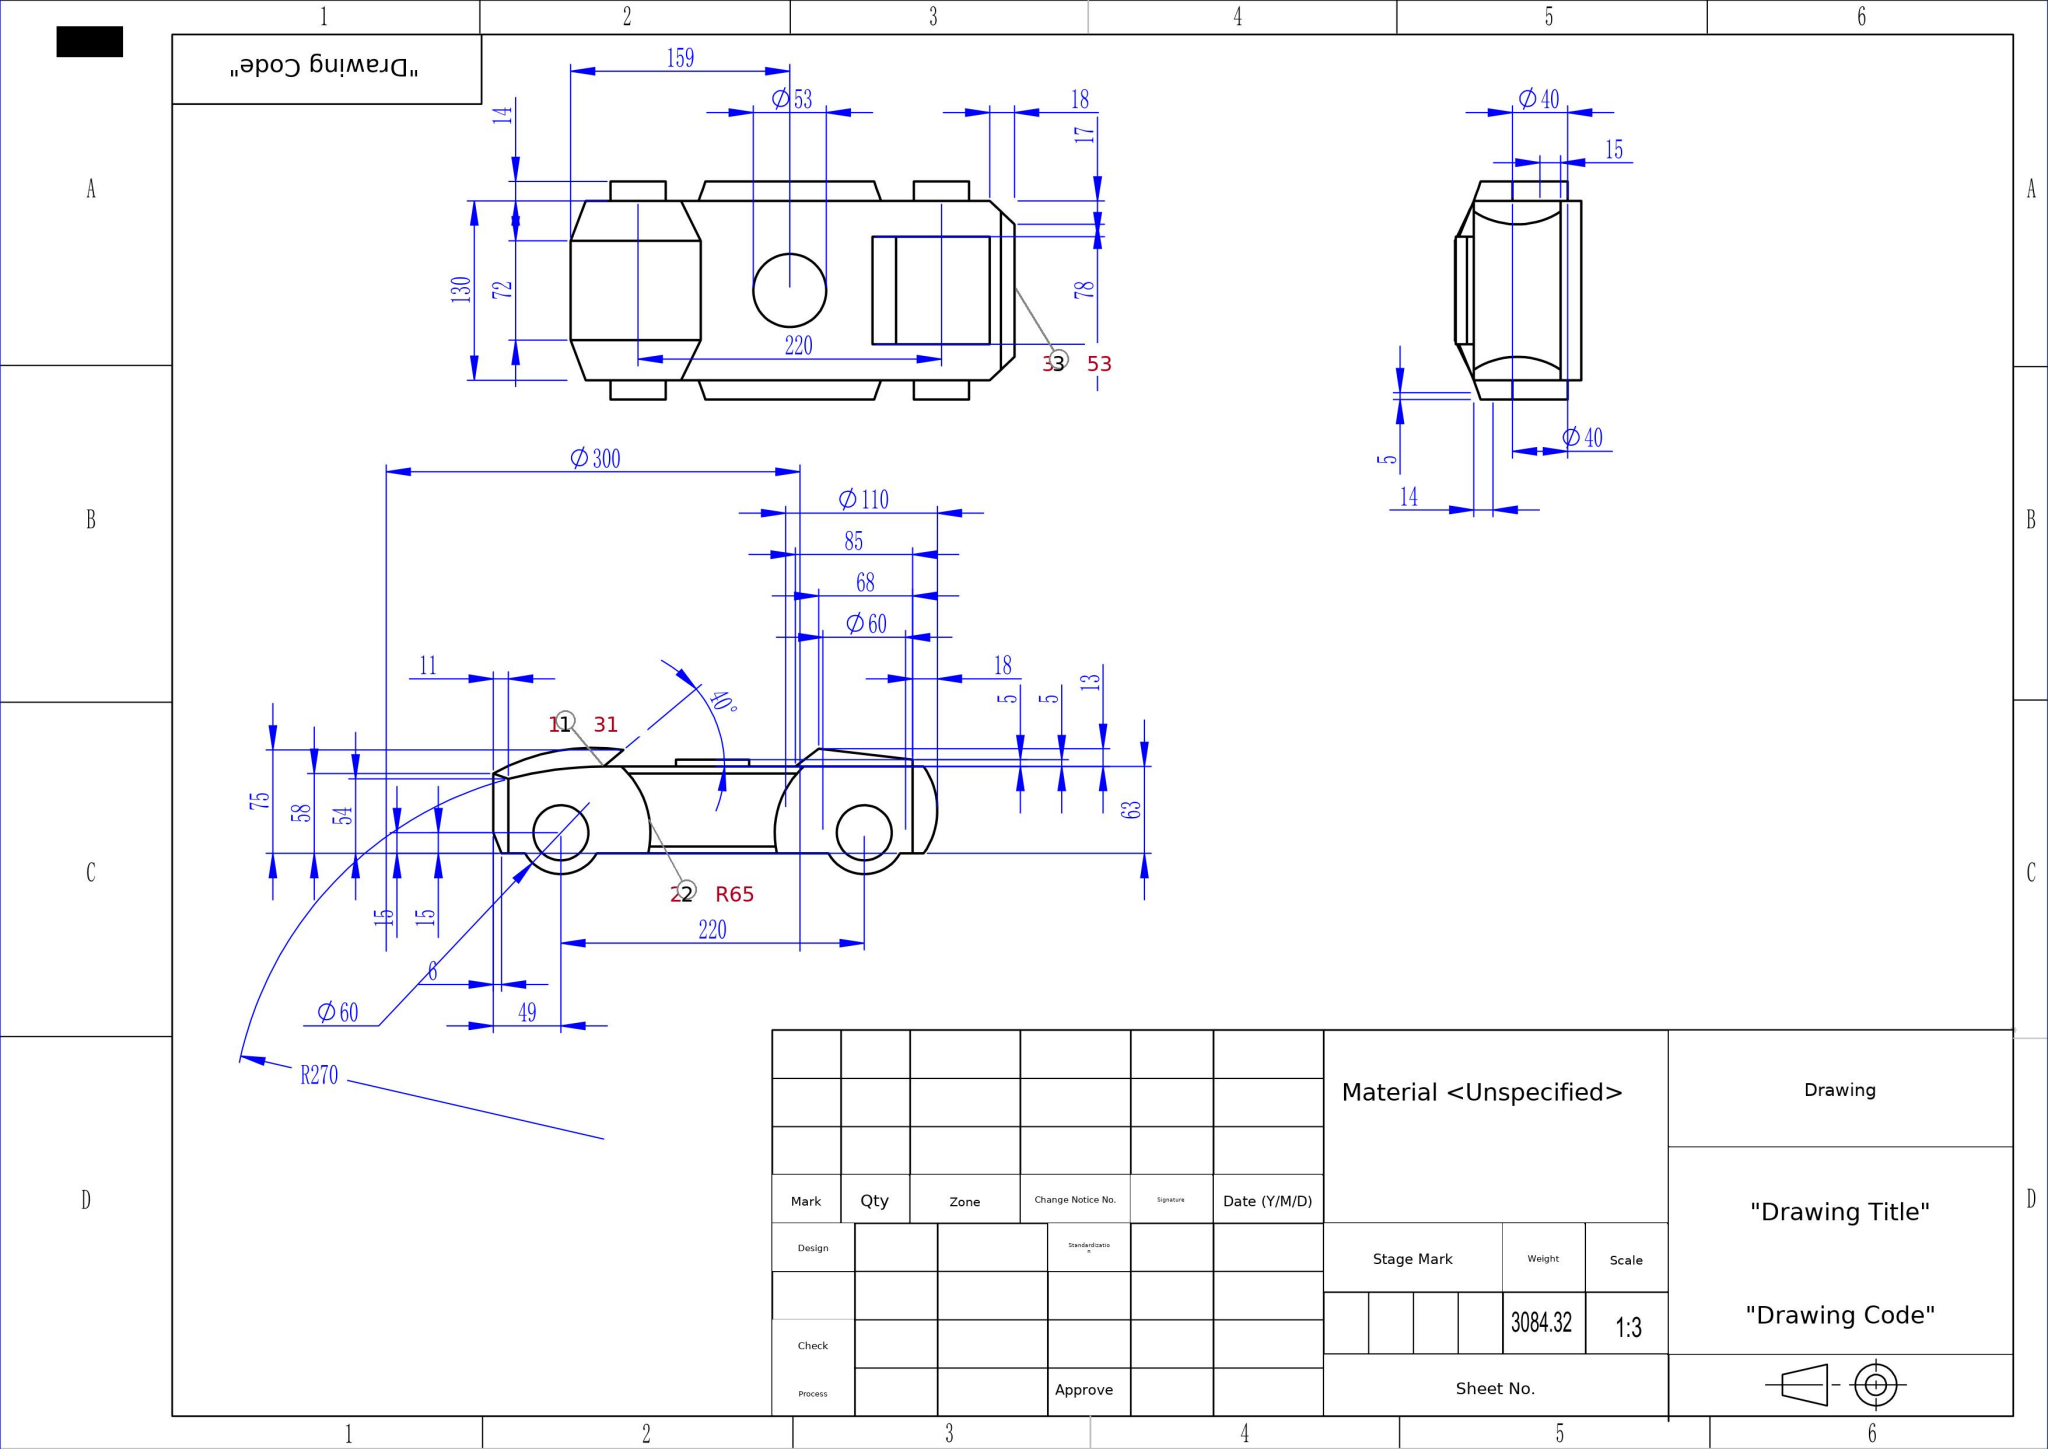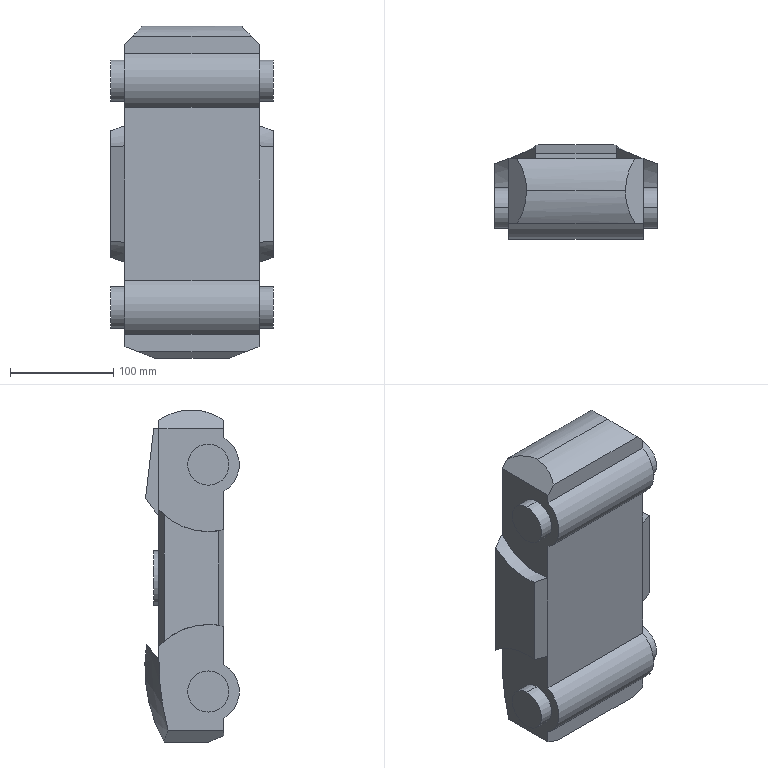Part | SolidWorks | mm | material Unspecified | 1 solid | 54 faces | box 158 x 91.63 x 322 mm | volume 3084326 mm3 | plane 31 | cylinder 21 | spline 2 | commonest cylinder face diameters 40 x8 130 x6 53 x2 110 x2 60 x2 300 x1